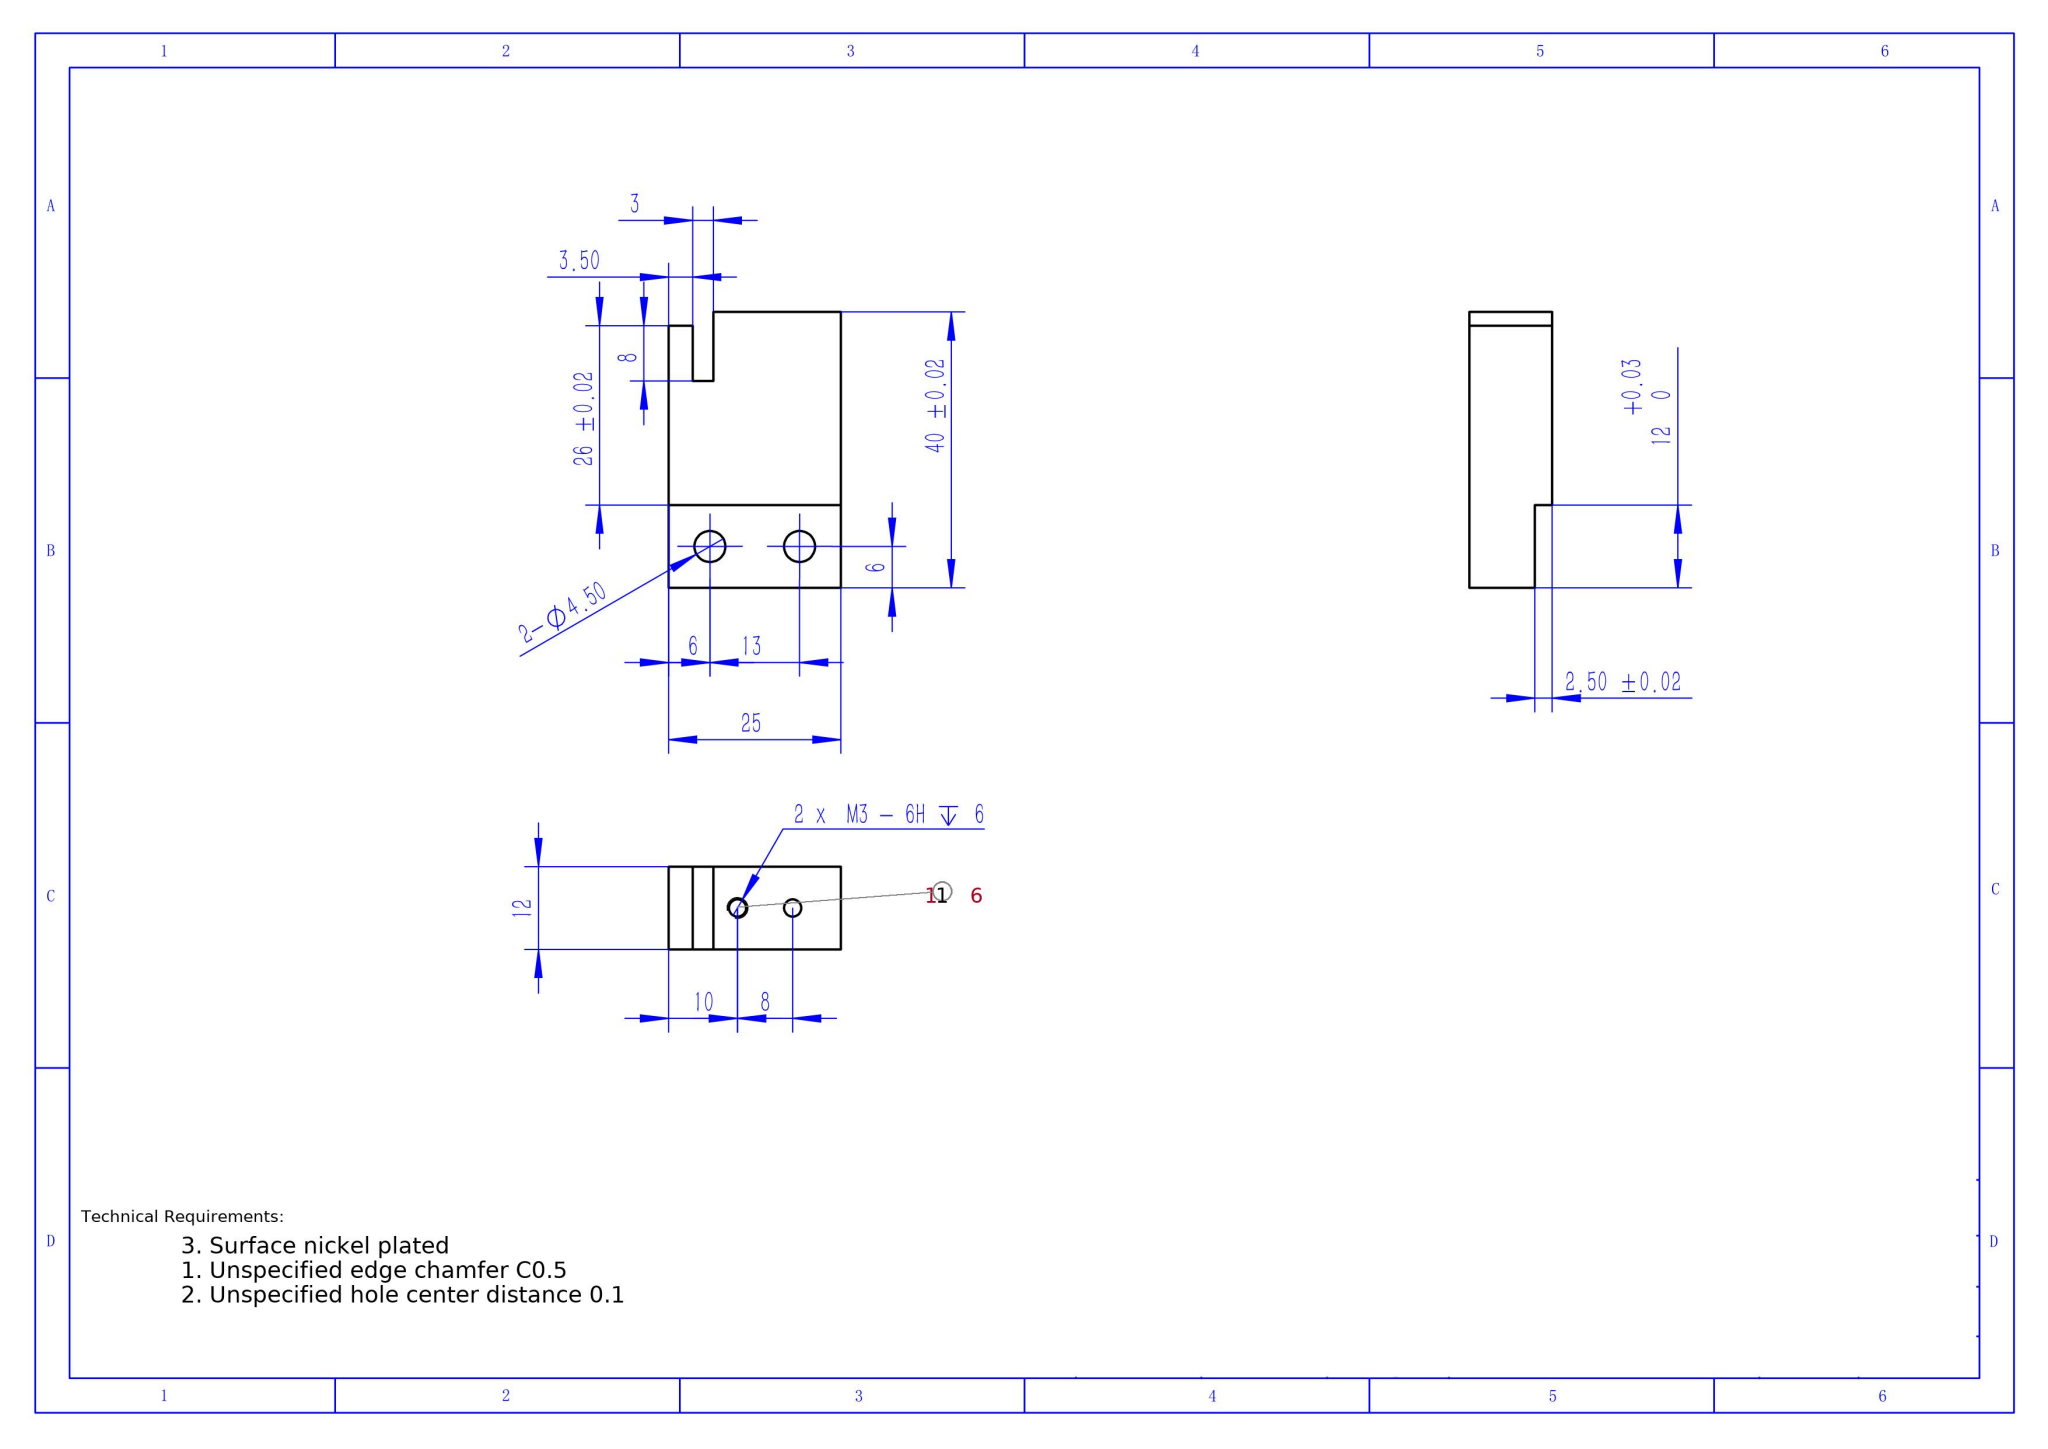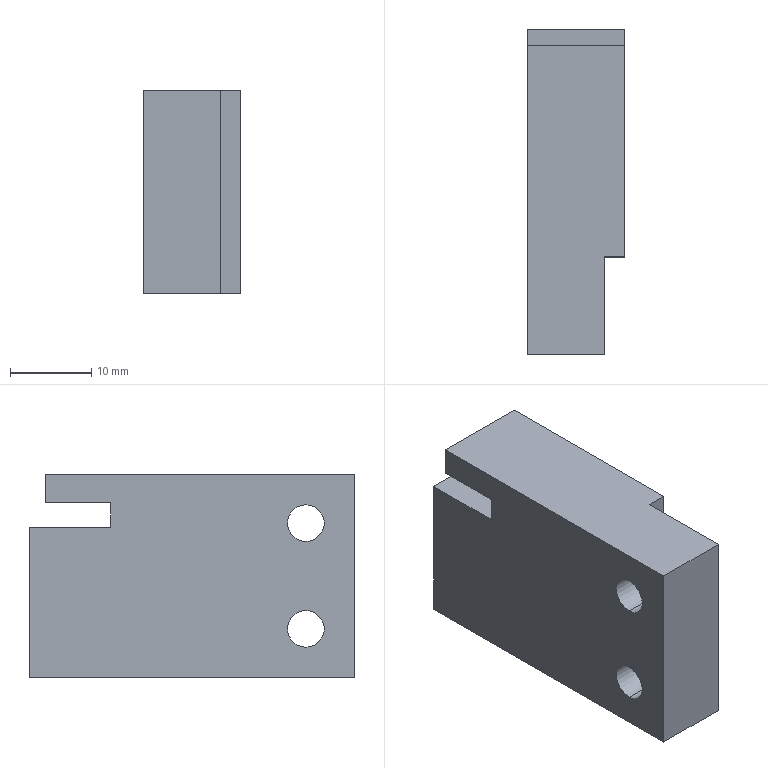Part | SolidWorks | mm | 1 solid | 24 faces | box 12 x 40 x 25 mm | volume 10418 mm3 | plane 12 | cylinder 8 | cone 4 | commonest cylinder face diameters 4.5 x4 2.5 x4
build123d program:
from build123d import *

# Parameters (mm, degrees)
SKETCH1_W             = 25
SKETCH1_H             = 40
BOSS_EXTRUDE1_DEPTH   = 6
M3_TAPPED_HOLE1_D     = 2.5
M3_TAPPED_HOLE1_DEPTH = 8.5
M3_TAPPED_HOLE1_TIP   = 0.7511
M4_CLEARANCE_HOLE_1_D = 4.5
SKETCH18_W            = 25
SKETCH18_H            = 12
CUT_EXTRUDE3_DEPTH    = 2.5
CUT_EXTRUDE4_DEPTH    = 27.462


with BuildPart() as part:
    # Sketch1 → Boss-Extrude1 (new, symmetric)
    with BuildSketch(Plane(origin=(0, 0, 0), x_dir=(0, 0, -1), z_dir=(1, 0, 0))):
        Rectangle(SKETCH1_W, SKETCH1_H)
    extrude(amount=BOSS_EXTRUDE1_DEPTH, both=True)

    # M3 Tapped Hole1
    with Locations(Plane(origin=(0, 20, 0), x_dir=(-1, 0, 0), z_dir=(0, 1, 0))):
        with Locations((0, 2.5), (0, -5.5)):
            Hole(M3_TAPPED_HOLE1_D / 2, depth=M3_TAPPED_HOLE1_DEPTH)
            with Locations((0, 0, -(M3_TAPPED_HOLE1_DEPTH + M3_TAPPED_HOLE1_TIP / 2))):  # 118° drill point
                Cone(0, M3_TAPPED_HOLE1_D / 2, M3_TAPPED_HOLE1_TIP, mode=Mode.SUBTRACT)

    # M4 Clearance Hole 1 (through all)
    with Locations(Plane.ZY.offset(6)):
        with Locations((-6.5, -14), (6.5, -14)):
            Hole(M4_CLEARANCE_HOLE_1_D / 2)

    # Sketch18 → Cut-Extrude3 (cut)
    with BuildSketch(Plane(origin=(6, 0, 0), x_dir=(0, 0, -1), z_dir=(1, 0, 0))):
        with Locations((0, -14)):
            Rectangle(SKETCH18_W, SKETCH18_H)
    extrude(amount=-CUT_EXTRUDE3_DEPTH, mode=Mode.SUBTRACT)

    # Sketch19 → Cut-Extrude4 (cut, through all)
    with BuildSketch(Plane.ZY.offset(6)):
        Polygon((12.5, 20), (12.5, 18), (9, 18), (9, 10), (6, 10), (6, 20), align=None)
    extrude(amount=-CUT_EXTRUDE4_DEPTH, mode=Mode.SUBTRACT)


solid = part.part
STEP:
#1=CARTESIAN_POINT('',(3.5,-14.,-4.25));
#2=VERTEX_POINT('',#1);
#3=CARTESIAN_POINT('',(3.5,-14.,-8.75));
#4=VERTEX_POINT('',#3);
#5=CARTESIAN_POINT('',(3.5,-14.,-6.5));
#6=DIRECTION('',(1.,0.,0.));
#7=DIRECTION('',(0.,0.,1.));
#8=AXIS2_PLACEMENT_3D('',#5,#6,#7);
#9=CIRCLE('',#8,2.25);
#10=EDGE_CURVE('',#2,#4,#9,.T.);
#11=ORIENTED_EDGE('',*,*,#10,.T.);
#12=CARTESIAN_POINT('',(-6.,-14.,-8.75));
#13=VERTEX_POINT('',#12);
#14=CARTESIAN_POINT('',(-6.,-14.,-8.75));
#15=DIRECTION('',(-1.,0.,0.));
#16=VECTOR('',#15,1000.);
#17=LINE('',#14,#16);
#18=EDGE_CURVE('',#4,#13,#17,.T.);
#19=ORIENTED_EDGE('',*,*,#18,.T.);
#20=CARTESIAN_POINT('',(-6.,-14.,-4.25));
#21=VERTEX_POINT('',#20);
#22=CARTESIAN_POINT('',(-6.,-14.,-6.5));
#23=DIRECTION('',(-1.,0.,0.));
#24=DIRECTION('',(0.,0.,1.));
#25=AXIS2_PLACEMENT_3D('',#22,#23,#24);
#26=CIRCLE('',#25,2.25);
#27=EDGE_CURVE('',#13,#21,#26,.T.);
#28=ORIENTED_EDGE('',*,*,#27,.T.);
#29=CARTESIAN_POINT('',(-6.,-14.,-4.25));
#30=DIRECTION('',(-1.,0.,0.));
#31=VECTOR('',#30,1000.);
#32=LINE('',#29,#31);
#33=EDGE_CURVE('',#2,#21,#32,.T.);
#34=ORIENTED_EDGE('',*,*,#33,.F.);
#35=EDGE_LOOP('',(#11,#19,#28,#34));
#36=FACE_OUTER_BOUND('',#35,.T.);
#37=CARTESIAN_POINT('',(-6.,-14.,-6.5));
#38=DIRECTION('',(-1.,0.,0.));
#39=DIRECTION('',(0.,0.,1.));
#40=AXIS2_PLACEMENT_3D('',#37,#38,#39);
#41=CYLINDRICAL_SURFACE('',#40,2.25);
#42=ADVANCED_FACE('',(#36),#41,.F.);
#43=CARTESIAN_POINT('',(3.5,-14.,8.75));
#44=VERTEX_POINT('',#43);
#45=CARTESIAN_POINT('',(3.5,-14.,4.25));
#46=VERTEX_POINT('',#45);
#47=CARTESIAN_POINT('',(3.5,-14.,6.5));
#48=DIRECTION('',(1.,0.,0.));
#49=DIRECTION('',(0.,0.,1.));
#50=AXIS2_PLACEMENT_3D('',#47,#48,#49);
#51=CIRCLE('',#50,2.25);
#52=EDGE_CURVE('',#44,#46,#51,.T.);
#53=ORIENTED_EDGE('',*,*,#52,.T.);
#54=CARTESIAN_POINT('',(-6.,-14.,4.25));
#55=VERTEX_POINT('',#54);
#56=CARTESIAN_POINT('',(-6.,-14.,4.25));
#57=DIRECTION('',(-1.,0.,0.));
#58=VECTOR('',#57,1000.);
#59=LINE('',#56,#58);
#60=EDGE_CURVE('',#46,#55,#59,.T.);
#61=ORIENTED_EDGE('',*,*,#60,.T.);
#62=CARTESIAN_POINT('',(-6.,-14.,8.75));
#63=VERTEX_POINT('',#62);
#64=CARTESIAN_POINT('',(-6.,-14.,6.5));
#65=DIRECTION('',(-1.,0.,0.));
#66=DIRECTION('',(0.,0.,1.));
#67=AXIS2_PLACEMENT_3D('',#64,#65,#66);
#68=CIRCLE('',#67,2.25);
#69=EDGE_CURVE('',#55,#63,#68,.T.);
#70=ORIENTED_EDGE('',*,*,#69,.T.);
#71=CARTESIAN_POINT('',(-6.,-14.,8.75));
#72=DIRECTION('',(-1.,0.,0.));
#73=VECTOR('',#72,1000.);
#74=LINE('',#71,#73);
#75=EDGE_CURVE('',#44,#63,#74,.T.);
#76=ORIENTED_EDGE('',*,*,#75,.F.);
#77=EDGE_LOOP('',(#53,#61,#70,#76));
#78=FACE_OUTER_BOUND('',#77,.T.);
#79=CARTESIAN_POINT('',(-6.,-14.,6.5));
#80=DIRECTION('',(-1.,0.,0.));
#81=DIRECTION('',(0.,0.,1.));
#82=AXIS2_PLACEMENT_3D('',#79,#80,#81);
#83=CYLINDRICAL_SURFACE('',#82,2.25);
#84=ADVANCED_FACE('',(#78),#83,.F.);
#85=CARTESIAN_POINT('',(0.,11.5,1.25));
#86=VERTEX_POINT('',#85);
#87=CARTESIAN_POINT('',(0.,11.5,3.75));
#88=VERTEX_POINT('',#87);
#89=CARTESIAN_POINT('',(0.,11.5,2.5));
#90=DIRECTION('',(0.,1.,0.));
#91=DIRECTION('',(0.,0.,1.));
#92=AXIS2_PLACEMENT_3D('',#89,#90,#91);
#93=CIRCLE('',#92,1.25);
#94=EDGE_CURVE('',#86,#88,#93,.T.);
#95=ORIENTED_EDGE('',*,*,#94,.F.);
#96=CARTESIAN_POINT('',(0.,20.,1.25));
#97=VERTEX_POINT('',#96);
#98=CARTESIAN_POINT('',(0.,20.,1.25));
#99=DIRECTION('',(0.,1.,0.));
#100=VECTOR('',#99,1000.);
#101=LINE('',#98,#100);
#102=EDGE_CURVE('',#86,#97,#101,.T.);
#103=ORIENTED_EDGE('',*,*,#102,.T.);
#104=CARTESIAN_POINT('',(0.,20.,3.75));
#105=VERTEX_POINT('',#104);
#106=CARTESIAN_POINT('',(0.,20.,2.5));
#107=DIRECTION('',(0.,1.,0.));
#108=DIRECTION('',(0.,0.,1.));
#109=AXIS2_PLACEMENT_3D('',#106,#107,#108);
#110=CIRCLE('',#109,1.25);
#111=EDGE_CURVE('',#97,#105,#110,.T.);
#112=ORIENTED_EDGE('',*,*,#111,.T.);
#113=CARTESIAN_POINT('',(0.,20.,3.75));
#114=DIRECTION('',(0.,1.,0.));
#115=VECTOR('',#114,1000.);
#116=LINE('',#113,#115);
#117=EDGE_CURVE('',#88,#105,#116,.T.);
#118=ORIENTED_EDGE('',*,*,#117,.F.);
#119=EDGE_LOOP('',(#95,#103,#112,#118));
#120=FACE_OUTER_BOUND('',#119,.T.);
#121=CARTESIAN_POINT('',(0.,20.,2.5));
#122=DIRECTION('',(0.,1.,0.));
#123=DIRECTION('',(0.,0.,1.));
#124=AXIS2_PLACEMENT_3D('',#121,#122,#123);
#125=CYLINDRICAL_SURFACE('',#124,1.25);
#126=ADVANCED_FACE('',(#120),#125,.F.);
#127=CARTESIAN_POINT('',(-0.,10.749,2.5));
#128=VERTEX_POINT('',#127);
#129=CARTESIAN_POINT('',(0.,11.5,3.75));
#130=DIRECTION('',(0.,0.515,0.8572));
#131=VECTOR('',#130,1000.);
#132=LINE('',#129,#131);
#133=EDGE_CURVE('',#128,#88,#132,.T.);
#134=ORIENTED_EDGE('',*,*,#133,.F.);
#135=CARTESIAN_POINT('',(0.,11.5,1.25));
#136=DIRECTION('',(0.,0.515,-0.8572));
#137=VECTOR('',#136,1000.);
#138=LINE('',#135,#137);
#139=EDGE_CURVE('',#128,#86,#138,.T.);
#140=ORIENTED_EDGE('',*,*,#139,.T.);
#141=ORIENTED_EDGE('',*,*,#94,.T.);
#142=EDGE_LOOP('',(#134,#140,#141));
#143=FACE_OUTER_BOUND('',#142,.T.);
#144=CARTESIAN_POINT('',(0.,11.5,2.5));
#145=DIRECTION('',(0.,1.,0.));
#146=DIRECTION('',(0.,0.,1.));
#147=AXIS2_PLACEMENT_3D('',#144,#145,#146);
#148=CONICAL_SURFACE('',#147,1.25,1.03);
#149=ADVANCED_FACE('',(#143),#148,.F.);
#150=CARTESIAN_POINT('',(0.,11.5,-6.75));
#151=VERTEX_POINT('',#150);
#152=CARTESIAN_POINT('',(0.,11.5,-4.25));
#153=VERTEX_POINT('',#152);
#154=CARTESIAN_POINT('',(0.,11.5,-5.5));
#155=DIRECTION('',(0.,1.,0.));
#156=DIRECTION('',(0.,0.,1.));
#157=AXIS2_PLACEMENT_3D('',#154,#155,#156);
#158=CIRCLE('',#157,1.25);
#159=EDGE_CURVE('',#151,#153,#158,.T.);
#160=ORIENTED_EDGE('',*,*,#159,.F.);
#161=CARTESIAN_POINT('',(0.,20.,-6.75));
#162=VERTEX_POINT('',#161);
#163=CARTESIAN_POINT('',(0.,20.,-6.75));
#164=DIRECTION('',(0.,1.,0.));
#165=VECTOR('',#164,1000.);
#166=LINE('',#163,#165);
#167=EDGE_CURVE('',#151,#162,#166,.T.);
#168=ORIENTED_EDGE('',*,*,#167,.T.);
#169=CARTESIAN_POINT('',(0.,20.,-4.25));
#170=VERTEX_POINT('',#169);
#171=CARTESIAN_POINT('',(0.,20.,-5.5));
#172=DIRECTION('',(0.,1.,0.));
#173=DIRECTION('',(0.,0.,1.));
#174=AXIS2_PLACEMENT_3D('',#171,#172,#173);
#175=CIRCLE('',#174,1.25);
#176=EDGE_CURVE('',#162,#170,#175,.T.);
#177=ORIENTED_EDGE('',*,*,#176,.T.);
#178=CARTESIAN_POINT('',(0.,20.,-4.25));
#179=DIRECTION('',(0.,1.,0.));
#180=VECTOR('',#179,1000.);
#181=LINE('',#178,#180);
#182=EDGE_CURVE('',#153,#170,#181,.T.);
#183=ORIENTED_EDGE('',*,*,#182,.F.);
#184=EDGE_LOOP('',(#160,#168,#177,#183));
#185=FACE_OUTER_BOUND('',#184,.T.);
#186=CARTESIAN_POINT('',(0.,20.,-5.5));
#187=DIRECTION('',(0.,1.,0.));
#188=DIRECTION('',(0.,0.,1.));
#189=AXIS2_PLACEMENT_3D('',#186,#187,#188);
#190=CYLINDRICAL_SURFACE('',#189,1.25);
#191=ADVANCED_FACE('',(#185),#190,.F.);
#192=CARTESIAN_POINT('',(-0.,10.749,-5.5));
#193=VERTEX_POINT('',#192);
#194=CARTESIAN_POINT('',(0.,11.5,-4.25));
#195=DIRECTION('',(0.,0.515,0.8572));
#196=VECTOR('',#195,1000.);
#197=LINE('',#194,#196);
#198=EDGE_CURVE('',#193,#153,#197,.T.);
#199=ORIENTED_EDGE('',*,*,#198,.F.);
#200=CARTESIAN_POINT('',(0.,11.5,-6.75));
#201=DIRECTION('',(0.,0.515,-0.8572));
#202=VECTOR('',#201,1000.);
#203=LINE('',#200,#202);
#204=EDGE_CURVE('',#193,#151,#203,.T.);
#205=ORIENTED_EDGE('',*,*,#204,.T.);
#206=ORIENTED_EDGE('',*,*,#159,.T.);
#207=EDGE_LOOP('',(#199,#205,#206));
#208=FACE_OUTER_BOUND('',#207,.T.);
#209=CARTESIAN_POINT('',(0.,11.5,-5.5));
#210=DIRECTION('',(0.,1.,0.));
#211=DIRECTION('',(0.,0.,1.));
#212=AXIS2_PLACEMENT_3D('',#209,#210,#211);
#213=CONICAL_SURFACE('',#212,1.25,1.03);
#214=ADVANCED_FACE('',(#208),#213,.F.);
#215=CARTESIAN_POINT('',(6.,-8.,-12.5));
#216=VERTEX_POINT('',#215);
#217=CARTESIAN_POINT('',(6.,20.,-12.5));
#218=VERTEX_POINT('',#217);
#219=CARTESIAN_POINT('',(6.,20.,-12.5));
#220=DIRECTION('',(0.,1.,0.));
#221=VECTOR('',#220,1000.);
#222=LINE('',#219,#221);
#223=EDGE_CURVE('',#216,#218,#222,.T.);
#224=ORIENTED_EDGE('',*,*,#223,.F.);
#225=CARTESIAN_POINT('',(3.5,-8.,-12.5));
#226=VERTEX_POINT('',#225);
#227=CARTESIAN_POINT('',(3.5,-8.,-12.5));
#228=DIRECTION('',(1.,0.,0.));
#229=VECTOR('',#228,1000.);
#230=LINE('',#227,#229);
#231=EDGE_CURVE('',#226,#216,#230,.T.);
#232=ORIENTED_EDGE('',*,*,#231,.F.);
#233=CARTESIAN_POINT('',(3.5,-20.,-12.5));
#234=VERTEX_POINT('',#233);
#235=CARTESIAN_POINT('',(3.5,-20.,-12.5));
#236=DIRECTION('',(0.,1.,0.));
#237=VECTOR('',#236,1000.);
#238=LINE('',#235,#237);
#239=EDGE_CURVE('',#234,#226,#238,.T.);
#240=ORIENTED_EDGE('',*,*,#239,.F.);
#241=CARTESIAN_POINT('',(-6.,-20.,-12.5));
#242=VERTEX_POINT('',#241);
#243=CARTESIAN_POINT('',(6.,-20.,-12.5));
#244=DIRECTION('',(-1.,0.,0.));
#245=VECTOR('',#244,1000.);
#246=LINE('',#243,#245);
#247=EDGE_CURVE('',#234,#242,#246,.T.);
#248=ORIENTED_EDGE('',*,*,#247,.T.);
#249=CARTESIAN_POINT('',(-6.,20.,-12.5));
#250=VERTEX_POINT('',#249);
#251=CARTESIAN_POINT('',(-6.,20.,-12.5));
#252=DIRECTION('',(0.,1.,0.));
#253=VECTOR('',#252,1000.);
#254=LINE('',#251,#253);
#255=EDGE_CURVE('',#242,#250,#254,.T.);
#256=ORIENTED_EDGE('',*,*,#255,.T.);
#257=CARTESIAN_POINT('',(6.,20.,-12.5));
#258=DIRECTION('',(-1.,0.,0.));
#259=VECTOR('',#258,1000.);
#260=LINE('',#257,#259);
#261=EDGE_CURVE('',#218,#250,#260,.T.);
#262=ORIENTED_EDGE('',*,*,#261,.F.);
#263=EDGE_LOOP('',(#224,#232,#240,#248,#256,#262));
#264=FACE_OUTER_BOUND('',#263,.T.);
#265=CARTESIAN_POINT('',(6.,20.,-12.5));
#266=DIRECTION('',(0.,-0.,1.));
#267=DIRECTION('',(0.,-1.,-0.));
#268=AXIS2_PLACEMENT_3D('',#265,#266,#267);
#269=PLANE('',#268);
#270=ADVANCED_FACE('',(#264),#269,.F.);
#271=CARTESIAN_POINT('',(0.,20.,2.5));
#272=DIRECTION('',(0.,1.,0.));
#273=DIRECTION('',(0.,0.,1.));
#274=AXIS2_PLACEMENT_3D('',#271,#272,#273);
#275=CIRCLE('',#274,1.25);
#276=EDGE_CURVE('',#105,#97,#275,.T.);
#277=ORIENTED_EDGE('',*,*,#276,.F.);
#278=ORIENTED_EDGE('',*,*,#111,.F.);
#279=EDGE_LOOP('',(#277,#278));
#280=FACE_BOUND('',#279,.T.);
#281=CARTESIAN_POINT('',(0.,20.,-5.5));
#282=DIRECTION('',(0.,1.,0.));
#283=DIRECTION('',(0.,0.,1.));
#284=AXIS2_PLACEMENT_3D('',#281,#282,#283);
#285=CIRCLE('',#284,1.25);
#286=EDGE_CURVE('',#170,#162,#285,.T.);
#287=ORIENTED_EDGE('',*,*,#286,.F.);
#288=ORIENTED_EDGE('',*,*,#176,.F.);
#289=EDGE_LOOP('',(#287,#288));
#290=FACE_BOUND('',#289,.T.);
#291=CARTESIAN_POINT('',(-6.,20.,6.));
#292=VERTEX_POINT('',#291);
#293=CARTESIAN_POINT('',(-6.,20.,12.5));
#294=DIRECTION('',(0.,0.,1.));
#295=VECTOR('',#294,1000.);
#296=LINE('',#293,#295);
#297=EDGE_CURVE('',#250,#292,#296,.T.);
#298=ORIENTED_EDGE('',*,*,#297,.T.);
#299=CARTESIAN_POINT('',(6.,20.,6.));
#300=VERTEX_POINT('',#299);
#301=CARTESIAN_POINT('',(6.,20.,6.));
#302=DIRECTION('',(-1.,0.,0.));
#303=VECTOR('',#302,1000.);
#304=LINE('',#301,#303);
#305=EDGE_CURVE('',#300,#292,#304,.T.);
#306=ORIENTED_EDGE('',*,*,#305,.F.);
#307=CARTESIAN_POINT('',(6.,20.,12.5));
#308=DIRECTION('',(0.,0.,1.));
#309=VECTOR('',#308,1000.);
#310=LINE('',#307,#309);
#311=EDGE_CURVE('',#218,#300,#310,.T.);
#312=ORIENTED_EDGE('',*,*,#311,.F.);
#313=ORIENTED_EDGE('',*,*,#261,.T.);
#314=EDGE_LOOP('',(#298,#306,#312,#313));
#315=FACE_OUTER_BOUND('',#314,.T.);
#316=CARTESIAN_POINT('',(6.,20.,12.5));
#317=DIRECTION('',(0.,-1.,0.));
#318=DIRECTION('',(0.,0.,-1.));
#319=AXIS2_PLACEMENT_3D('',#316,#317,#318);
#320=PLANE('',#319);
#321=ADVANCED_FACE('',(#280,#290,#315),#320,.F.);
#322=CARTESIAN_POINT('',(6.,18.,12.5));
#323=VERTEX_POINT('',#322);
#324=CARTESIAN_POINT('',(6.,-8.,12.5));
#325=VERTEX_POINT('',#324);
#326=CARTESIAN_POINT('',(6.,20.,12.5));
#327=DIRECTION('',(0.,-1.,-0.));
#328=VECTOR('',#327,1000.);
#329=LINE('',#326,#328);
#330=EDGE_CURVE('',#323,#325,#329,.T.);
#331=ORIENTED_EDGE('',*,*,#330,.F.);
#332=CARTESIAN_POINT('',(-6.,18.,12.5));
#333=VERTEX_POINT('',#332);
#334=CARTESIAN_POINT('',(6.,18.,12.5));
#335=DIRECTION('',(-1.,0.,0.));
#336=VECTOR('',#335,1000.);
#337=LINE('',#334,#336);
#338=EDGE_CURVE('',#323,#333,#337,.T.);
#339=ORIENTED_EDGE('',*,*,#338,.T.);
#340=CARTESIAN_POINT('',(-6.,-20.,12.5));
#341=VERTEX_POINT('',#340);
#342=CARTESIAN_POINT('',(-6.,20.,12.5));
#343=DIRECTION('',(0.,-1.,-0.));
#344=VECTOR('',#343,1000.);
#345=LINE('',#342,#344);
#346=EDGE_CURVE('',#333,#341,#345,.T.);
#347=ORIENTED_EDGE('',*,*,#346,.T.);
#348=CARTESIAN_POINT('',(3.5,-20.,12.5));
#349=VERTEX_POINT('',#348);
#350=CARTESIAN_POINT('',(6.,-20.,12.5));
#351=DIRECTION('',(-1.,0.,0.));
#352=VECTOR('',#351,1000.);
#353=LINE('',#350,#352);
#354=EDGE_CURVE('',#349,#341,#353,.T.);
#355=ORIENTED_EDGE('',*,*,#354,.F.);
#356=CARTESIAN_POINT('',(3.5,-8.,12.5));
#357=VERTEX_POINT('',#356);
#358=CARTESIAN_POINT('',(3.5,-20.,12.5));
#359=DIRECTION('',(0.,-1.,0.));
#360=VECTOR('',#359,1000.);
#361=LINE('',#358,#360);
#362=EDGE_CURVE('',#357,#349,#361,.T.);
#363=ORIENTED_EDGE('',*,*,#362,.F.);
#364=CARTESIAN_POINT('',(3.5,-8.,12.5));
#365=DIRECTION('',(1.,0.,0.));
#366=VECTOR('',#365,1000.);
#367=LINE('',#364,#366);
#368=EDGE_CURVE('',#357,#325,#367,.T.);
#369=ORIENTED_EDGE('',*,*,#368,.T.);
#370=EDGE_LOOP('',(#331,#339,#347,#355,#363,#369));
#371=FACE_OUTER_BOUND('',#370,.T.);
#372=CARTESIAN_POINT('',(6.,20.,12.5));
#373=DIRECTION('',(0.,0.,-1.));
#374=DIRECTION('',(0.,1.,0.));
#375=AXIS2_PLACEMENT_3D('',#372,#373,#374);
#376=PLANE('',#375);
#377=ADVANCED_FACE('',(#371),#376,.F.);
#378=ORIENTED_EDGE('',*,*,#247,.F.);
#379=CARTESIAN_POINT('',(3.5,-20.,12.5));
#380=DIRECTION('',(0.,0.,-1.));
#381=VECTOR('',#380,1000.);
#382=LINE('',#379,#381);
#383=EDGE_CURVE('',#349,#234,#382,.T.);
#384=ORIENTED_EDGE('',*,*,#383,.F.);
#385=ORIENTED_EDGE('',*,*,#354,.T.);
#386=CARTESIAN_POINT('',(-6.,-20.,12.5));
#387=DIRECTION('',(0.,0.,-1.));
#388=VECTOR('',#387,1000.);
#389=LINE('',#386,#388);
#390=EDGE_CURVE('',#341,#242,#389,.T.);
#391=ORIENTED_EDGE('',*,*,#390,.T.);
#392=EDGE_LOOP('',(#378,#384,#385,#391));
#393=FACE_OUTER_BOUND('',#392,.T.);
#394=CARTESIAN_POINT('',(6.,-20.,12.5));
#395=DIRECTION('',(0.,1.,0.));
#396=DIRECTION('',(0.,0.,1.));
#397=AXIS2_PLACEMENT_3D('',#394,#395,#396);
#398=PLANE('',#397);
#399=ADVANCED_FACE('',(#393),#398,.F.);
#400=CARTESIAN_POINT('',(6.,18.,9.));
#401=VERTEX_POINT('',#400);
#402=CARTESIAN_POINT('',(6.,18.,12.5));
#403=DIRECTION('',(0.,0.,1.));
#404=VECTOR('',#403,1000.);
#405=LINE('',#402,#404);
#406=EDGE_CURVE('',#401,#323,#405,.T.);
#407=ORIENTED_EDGE('',*,*,#406,.T.);
#408=ORIENTED_EDGE('',*,*,#330,.T.);
#409=CARTESIAN_POINT('',(6.,-8.,12.5));
#410=DIRECTION('',(0.,0.,1.));
#411=VECTOR('',#410,1000.);
#412=LINE('',#409,#411);
#413=EDGE_CURVE('',#216,#325,#412,.T.);
#414=ORIENTED_EDGE('',*,*,#413,.F.);
#415=ORIENTED_EDGE('',*,*,#223,.T.);
#416=ORIENTED_EDGE('',*,*,#311,.T.);
#417=CARTESIAN_POINT('',(6.,10.,6.));
#418=VERTEX_POINT('',#417);
#419=CARTESIAN_POINT('',(6.,10.,6.));
#420=DIRECTION('',(0.,-1.,0.));
#421=VECTOR('',#420,1000.);
#422=LINE('',#419,#421);
#423=EDGE_CURVE('',#300,#418,#422,.T.);
#424=ORIENTED_EDGE('',*,*,#423,.T.);
#425=CARTESIAN_POINT('',(6.,10.,9.));
#426=VERTEX_POINT('',#425);
#427=CARTESIAN_POINT('',(6.,10.,9.));
#428=DIRECTION('',(0.,0.,1.));
#429=VECTOR('',#428,1000.);
#430=LINE('',#427,#429);
#431=EDGE_CURVE('',#418,#426,#430,.T.);
#432=ORIENTED_EDGE('',*,*,#431,.T.);
#433=CARTESIAN_POINT('',(6.,18.,9.));
#434=DIRECTION('',(0.,1.,-0.));
#435=VECTOR('',#434,1000.);
#436=LINE('',#433,#435);
#437=EDGE_CURVE('',#426,#401,#436,.T.);
#438=ORIENTED_EDGE('',*,*,#437,.T.);
#439=EDGE_LOOP('',(#407,#408,#414,#415,#416,#424,#432,#438));
#440=FACE_OUTER_BOUND('',#439,.T.);
#441=CARTESIAN_POINT('',(6.,-20.,-12.5));
#442=DIRECTION('',(1.,0.,0.));
#443=DIRECTION('',(0.,0.,-1.));
#444=AXIS2_PLACEMENT_3D('',#441,#442,#443);
#445=PLANE('',#444);
#446=ADVANCED_FACE('',(#440),#445,.T.);
#447=CARTESIAN_POINT('',(-6.,-14.,-6.5));
#448=DIRECTION('',(-1.,0.,0.));
#449=DIRECTION('',(0.,0.,1.));
#450=AXIS2_PLACEMENT_3D('',#447,#448,#449);
#451=CIRCLE('',#450,2.25);
#452=EDGE_CURVE('',#21,#13,#451,.T.);
#453=ORIENTED_EDGE('',*,*,#452,.F.);
#454=ORIENTED_EDGE('',*,*,#27,.F.);
#455=EDGE_LOOP('',(#453,#454));
#456=FACE_BOUND('',#455,.T.);
#457=CARTESIAN_POINT('',(-6.,-14.,6.5));
#458=DIRECTION('',(-1.,0.,0.));
#459=DIRECTION('',(0.,0.,1.));
#460=AXIS2_PLACEMENT_3D('',#457,#458,#459);
#461=CIRCLE('',#460,2.25);
#462=EDGE_CURVE('',#63,#55,#461,.T.);
#463=ORIENTED_EDGE('',*,*,#462,.F.);
#464=ORIENTED_EDGE('',*,*,#69,.F.);
#465=EDGE_LOOP('',(#463,#464));
#466=FACE_BOUND('',#465,.T.);
#467=ORIENTED_EDGE('',*,*,#346,.F.);
#468=CARTESIAN_POINT('',(-6.,18.,9.));
#469=VERTEX_POINT('',#468);
#470=CARTESIAN_POINT('',(-6.,18.,12.5));
#471=DIRECTION('',(0.,0.,1.));
#472=VECTOR('',#471,1000.);
#473=LINE('',#470,#472);
#474=EDGE_CURVE('',#469,#333,#473,.T.);
#475=ORIENTED_EDGE('',*,*,#474,.F.);
#476=CARTESIAN_POINT('',(-6.,10.,9.));
#477=VERTEX_POINT('',#476);
#478=CARTESIAN_POINT('',(-6.,18.,9.));
#479=DIRECTION('',(0.,1.,-0.));
#480=VECTOR('',#479,1000.);
#481=LINE('',#478,#480);
#482=EDGE_CURVE('',#477,#469,#481,.T.);
#483=ORIENTED_EDGE('',*,*,#482,.F.);
#484=CARTESIAN_POINT('',(-6.,10.,6.));
#485=VERTEX_POINT('',#484);
#486=CARTESIAN_POINT('',(-6.,10.,9.));
#487=DIRECTION('',(0.,0.,1.));
#488=VECTOR('',#487,1000.);
#489=LINE('',#486,#488);
#490=EDGE_CURVE('',#485,#477,#489,.T.);
#491=ORIENTED_EDGE('',*,*,#490,.F.);
#492=CARTESIAN_POINT('',(-6.,10.,6.));
#493=DIRECTION('',(0.,-1.,0.));
#494=VECTOR('',#493,1000.);
#495=LINE('',#492,#494);
#496=EDGE_CURVE('',#292,#485,#495,.T.);
#497=ORIENTED_EDGE('',*,*,#496,.F.);
#498=ORIENTED_EDGE('',*,*,#297,.F.);
#499=ORIENTED_EDGE('',*,*,#255,.F.);
#500=ORIENTED_EDGE('',*,*,#390,.F.);
#501=EDGE_LOOP('',(#467,#475,#483,#491,#497,#498,#499,#500));
#502=FACE_OUTER_BOUND('',#501,.T.);
#503=CARTESIAN_POINT('',(-6.,-20.,-12.5));
#504=DIRECTION('',(1.,0.,0.));
#505=DIRECTION('',(0.,0.,-1.));
#506=AXIS2_PLACEMENT_3D('',#503,#504,#505);
#507=PLANE('',#506);
#508=ADVANCED_FACE('',(#456,#466,#502),#507,.F.);
#509=ORIENTED_EDGE('',*,*,#204,.F.);
#510=ORIENTED_EDGE('',*,*,#198,.T.);
#511=CARTESIAN_POINT('',(0.,11.5,-5.5));
#512=DIRECTION('',(0.,1.,0.));
#513=DIRECTION('',(0.,0.,1.));
#514=AXIS2_PLACEMENT_3D('',#511,#512,#513);
#515=CIRCLE('',#514,1.25);
#516=EDGE_CURVE('',#153,#151,#515,.T.);
#517=ORIENTED_EDGE('',*,*,#516,.T.);
#518=EDGE_LOOP('',(#509,#510,#517));
#519=FACE_OUTER_BOUND('',#518,.T.);
#520=CARTESIAN_POINT('',(0.,11.5,-5.5));
#521=DIRECTION('',(0.,1.,0.));
#522=DIRECTION('',(0.,0.,1.));
#523=AXIS2_PLACEMENT_3D('',#520,#521,#522);
#524=CONICAL_SURFACE('',#523,1.25,1.03);
#525=ADVANCED_FACE('',(#519),#524,.F.);
#526=ORIENTED_EDGE('',*,*,#167,.F.);
#527=ORIENTED_EDGE('',*,*,#516,.F.);
#528=ORIENTED_EDGE('',*,*,#182,.T.);
#529=ORIENTED_EDGE('',*,*,#286,.T.);
#530=EDGE_LOOP('',(#526,#527,#528,#529));
#531=FACE_OUTER_BOUND('',#530,.T.);
#532=CARTESIAN_POINT('',(0.,20.,-5.5));
#533=DIRECTION('',(0.,1.,0.));
#534=DIRECTION('',(0.,0.,1.));
#535=AXIS2_PLACEMENT_3D('',#532,#533,#534);
#536=CYLINDRICAL_SURFACE('',#535,1.25);
#537=ADVANCED_FACE('',(#531),#536,.F.);
#538=ORIENTED_EDGE('',*,*,#139,.F.);
#539=ORIENTED_EDGE('',*,*,#133,.T.);
#540=CARTESIAN_POINT('',(0.,11.5,2.5));
#541=DIRECTION('',(0.,1.,0.));
#542=DIRECTION('',(0.,0.,1.));
#543=AXIS2_PLACEMENT_3D('',#540,#541,#542);
#544=CIRCLE('',#543,1.25);
#545=EDGE_CURVE('',#88,#86,#544,.T.);
#546=ORIENTED_EDGE('',*,*,#545,.T.);
#547=EDGE_LOOP('',(#538,#539,#546));
#548=FACE_OUTER_BOUND('',#547,.T.);
#549=CARTESIAN_POINT('',(0.,11.5,2.5));
#550=DIRECTION('',(0.,1.,0.));
#551=DIRECTION('',(0.,0.,1.));
#552=AXIS2_PLACEMENT_3D('',#549,#550,#551);
#553=CONICAL_SURFACE('',#552,1.25,1.03);
#554=ADVANCED_FACE('',(#548),#553,.F.);
#555=ORIENTED_EDGE('',*,*,#102,.F.);
#556=ORIENTED_EDGE('',*,*,#545,.F.);
#557=ORIENTED_EDGE('',*,*,#117,.T.);
#558=ORIENTED_EDGE('',*,*,#276,.T.);
#559=EDGE_LOOP('',(#555,#556,#557,#558));
#560=FACE_OUTER_BOUND('',#559,.T.);
#561=CARTESIAN_POINT('',(0.,20.,2.5));
#562=DIRECTION('',(0.,1.,0.));
#563=DIRECTION('',(0.,0.,1.));
#564=AXIS2_PLACEMENT_3D('',#561,#562,#563);
#565=CYLINDRICAL_SURFACE('',#564,1.25);
#566=ADVANCED_FACE('',(#560),#565,.F.);
#567=ORIENTED_EDGE('',*,*,#60,.F.);
#568=CARTESIAN_POINT('',(3.5,-14.,6.5));
#569=DIRECTION('',(1.,0.,0.));
#570=DIRECTION('',(0.,0.,1.));
#571=AXIS2_PLACEMENT_3D('',#568,#569,#570);
#572=CIRCLE('',#571,2.25);
#573=EDGE_CURVE('',#46,#44,#572,.T.);
#574=ORIENTED_EDGE('',*,*,#573,.T.);
#575=ORIENTED_EDGE('',*,*,#75,.T.);
#576=ORIENTED_EDGE('',*,*,#462,.T.);
#577=EDGE_LOOP('',(#567,#574,#575,#576));
#578=FACE_OUTER_BOUND('',#577,.T.);
#579=CARTESIAN_POINT('',(-6.,-14.,6.5));
#580=DIRECTION('',(-1.,0.,0.));
#581=DIRECTION('',(0.,0.,1.));
#582=AXIS2_PLACEMENT_3D('',#579,#580,#581);
#583=CYLINDRICAL_SURFACE('',#582,2.25);
#584=ADVANCED_FACE('',(#578),#583,.F.);
#585=ORIENTED_EDGE('',*,*,#18,.F.);
#586=CARTESIAN_POINT('',(3.5,-14.,-6.5));
#587=DIRECTION('',(1.,0.,0.));
#588=DIRECTION('',(0.,0.,1.));
#589=AXIS2_PLACEMENT_3D('',#586,#587,#588);
#590=CIRCLE('',#589,2.25);
#591=EDGE_CURVE('',#4,#2,#590,.T.);
#592=ORIENTED_EDGE('',*,*,#591,.T.);
#593=ORIENTED_EDGE('',*,*,#33,.T.);
#594=ORIENTED_EDGE('',*,*,#452,.T.);
#595=EDGE_LOOP('',(#585,#592,#593,#594));
#596=FACE_OUTER_BOUND('',#595,.T.);
#597=CARTESIAN_POINT('',(-6.,-14.,-6.5));
#598=DIRECTION('',(-1.,0.,0.));
#599=DIRECTION('',(0.,0.,1.));
#600=AXIS2_PLACEMENT_3D('',#597,#598,#599);
#601=CYLINDRICAL_SURFACE('',#600,2.25);
#602=ADVANCED_FACE('',(#596),#601,.F.);
#603=ORIENTED_EDGE('',*,*,#10,.F.);
#604=ORIENTED_EDGE('',*,*,#591,.F.);
#605=EDGE_LOOP('',(#603,#604));
#606=FACE_BOUND('',#605,.T.);
#607=ORIENTED_EDGE('',*,*,#362,.T.);
#608=ORIENTED_EDGE('',*,*,#383,.T.);
#609=ORIENTED_EDGE('',*,*,#239,.T.);
#610=CARTESIAN_POINT('',(3.5,-8.,12.5));
#611=DIRECTION('',(0.,0.,1.));
#612=VECTOR('',#611,1000.);
#613=LINE('',#610,#612);
#614=EDGE_CURVE('',#226,#357,#613,.T.);
#615=ORIENTED_EDGE('',*,*,#614,.T.);
#616=EDGE_LOOP('',(#607,#608,#609,#615));
#617=FACE_OUTER_BOUND('',#616,.T.);
#618=ORIENTED_EDGE('',*,*,#52,.F.);
#619=ORIENTED_EDGE('',*,*,#573,.F.);
#620=EDGE_LOOP('',(#618,#619));
#621=FACE_BOUND('',#620,.T.);
#622=CARTESIAN_POINT('',(3.5,0.,0.));
#623=DIRECTION('',(-1.,0.,0.));
#624=DIRECTION('',(0.,0.,1.));
#625=AXIS2_PLACEMENT_3D('',#622,#623,#624);
#626=PLANE('',#625);
#627=ADVANCED_FACE('',(#606,#617,#621),#626,.F.);
#628=ORIENTED_EDGE('',*,*,#413,.T.);
#629=ORIENTED_EDGE('',*,*,#368,.F.);
#630=ORIENTED_EDGE('',*,*,#614,.F.);
#631=ORIENTED_EDGE('',*,*,#231,.T.);
#632=EDGE_LOOP('',(#628,#629,#630,#631));
#633=FACE_OUTER_BOUND('',#632,.T.);
#634=CARTESIAN_POINT('',(3.5,-8.,12.5));
#635=DIRECTION('',(0.,1.,0.));
#636=DIRECTION('',(0.,0.,1.));
#637=AXIS2_PLACEMENT_3D('',#634,#635,#636);
#638=PLANE('',#637);
#639=ADVANCED_FACE('',(#633),#638,.F.);
#640=ORIENTED_EDGE('',*,*,#474,.T.);
#641=ORIENTED_EDGE('',*,*,#338,.F.);
#642=ORIENTED_EDGE('',*,*,#406,.F.);
#643=CARTESIAN_POINT('',(6.,18.,9.));
#644=DIRECTION('',(-1.,0.,0.));
#645=VECTOR('',#644,1000.);
#646=LINE('',#643,#645);
#647=EDGE_CURVE('',#401,#469,#646,.T.);
#648=ORIENTED_EDGE('',*,*,#647,.T.);
#649=EDGE_LOOP('',(#640,#641,#642,#648));
#650=FACE_OUTER_BOUND('',#649,.T.);
#651=CARTESIAN_POINT('',(6.,18.,12.5));
#652=DIRECTION('',(0.,-1.,0.));
#653=DIRECTION('',(0.,0.,-1.));
#654=AXIS2_PLACEMENT_3D('',#651,#652,#653);
#655=PLANE('',#654);
#656=ADVANCED_FACE('',(#650),#655,.F.);
#657=ORIENTED_EDGE('',*,*,#482,.T.);
#658=ORIENTED_EDGE('',*,*,#647,.F.);
#659=ORIENTED_EDGE('',*,*,#437,.F.);
#660=CARTESIAN_POINT('',(6.,10.,9.));
#661=DIRECTION('',(-1.,0.,0.));
#662=VECTOR('',#661,1000.);
#663=LINE('',#660,#662);
#664=EDGE_CURVE('',#426,#477,#663,.T.);
#665=ORIENTED_EDGE('',*,*,#664,.T.);
#666=EDGE_LOOP('',(#657,#658,#659,#665));
#667=FACE_OUTER_BOUND('',#666,.T.);
#668=CARTESIAN_POINT('',(6.,18.,9.));
#669=DIRECTION('',(0.,0.,1.));
#670=DIRECTION('',(0.,-1.,0.));
#671=AXIS2_PLACEMENT_3D('',#668,#669,#670);
#672=PLANE('',#671);
#673=ADVANCED_FACE('',(#667),#672,.F.);
#674=ORIENTED_EDGE('',*,*,#490,.T.);
#675=ORIENTED_EDGE('',*,*,#664,.F.);
#676=ORIENTED_EDGE('',*,*,#431,.F.);
#677=CARTESIAN_POINT('',(6.,10.,6.));
#678=DIRECTION('',(-1.,0.,0.));
#679=VECTOR('',#678,1000.);
#680=LINE('',#677,#679);
#681=EDGE_CURVE('',#418,#485,#680,.T.);
#682=ORIENTED_EDGE('',*,*,#681,.T.);
#683=EDGE_LOOP('',(#674,#675,#676,#682));
#684=FACE_OUTER_BOUND('',#683,.T.);
#685=CARTESIAN_POINT('',(6.,10.,9.));
#686=DIRECTION('',(0.,-1.,0.));
#687=DIRECTION('',(0.,0.,-1.));
#688=AXIS2_PLACEMENT_3D('',#685,#686,#687);
#689=PLANE('',#688);
#690=ADVANCED_FACE('',(#684),#689,.F.);
#691=ORIENTED_EDGE('',*,*,#496,.T.);
#692=ORIENTED_EDGE('',*,*,#681,.F.);
#693=ORIENTED_EDGE('',*,*,#423,.F.);
#694=ORIENTED_EDGE('',*,*,#305,.T.);
#695=EDGE_LOOP('',(#691,#692,#693,#694));
#696=FACE_OUTER_BOUND('',#695,.T.);
#697=CARTESIAN_POINT('',(6.,10.,6.));
#698=DIRECTION('',(0.,-0.,-1.));
#699=DIRECTION('',(0.,1.,-0.));
#700=AXIS2_PLACEMENT_3D('',#697,#698,#699);
#701=PLANE('',#700);
#702=ADVANCED_FACE('',(#696),#701,.F.);
#703=CLOSED_SHELL('',(#42,#84,#126,#149,#191,#214,#270,#321,#377,#399,#446,#508,#525,#537,#554,#566,#584,#602,#627,#639,#656,#673,#690,#702));
#704=MANIFOLD_SOLID_BREP('',#703);
#705=CARTESIAN_POINT('',(0.,0.,0.));
#706=DIRECTION('',(0.,0.,1.));
#707=DIRECTION('',(1.,0.,0.));
#708=AXIS2_PLACEMENT_3D('',#705,#706,#707);
#709=(LENGTH_UNIT()NAMED_UNIT(*)SI_UNIT(.MILLI.,.METRE.));
#710=UNCERTAINTY_MEASURE_WITH_UNIT(LENGTH_MEASURE(0.00001),#709,'','');
#711=(NAMED_UNIT(*)PLANE_ANGLE_UNIT()SI_UNIT($,.RADIAN.));
#712=(NAMED_UNIT(*)SI_UNIT($,.STERADIAN.)SOLID_ANGLE_UNIT());
#713=(GEOMETRIC_REPRESENTATION_CONTEXT(3)GLOBAL_UNCERTAINTY_ASSIGNED_CONTEXT((#710))GLOBAL_UNIT_ASSIGNED_CONTEXT((#709,#711,#712))REPRESENTATION_CONTEXT('',''));
#714=ADVANCED_BREP_SHAPE_REPRESENTATION('',(#704,#708),#713);